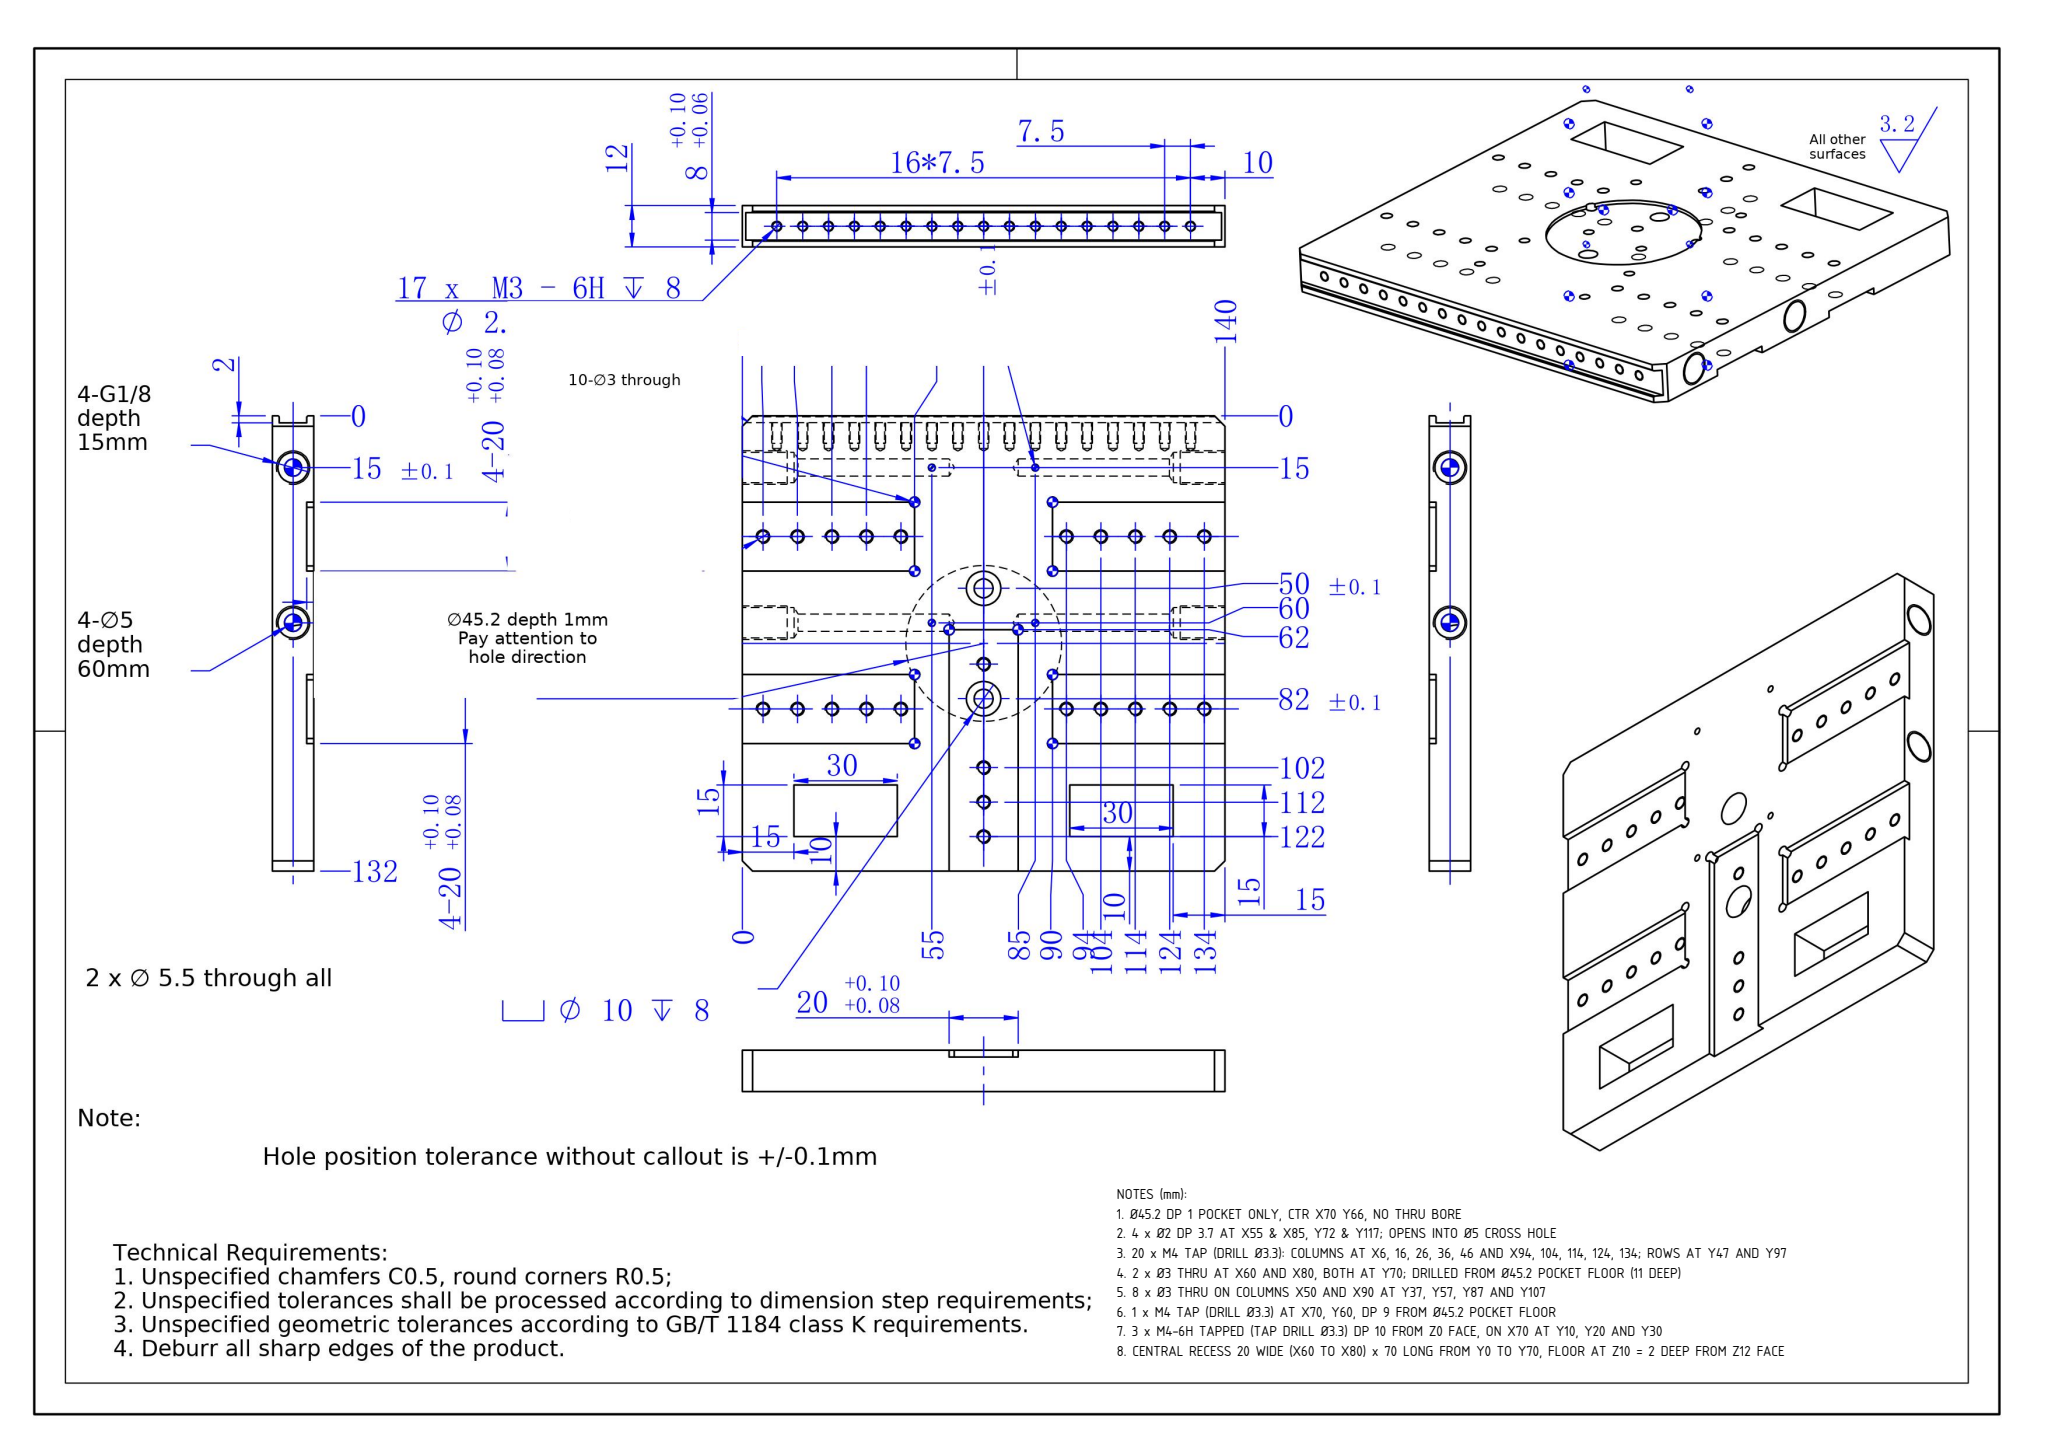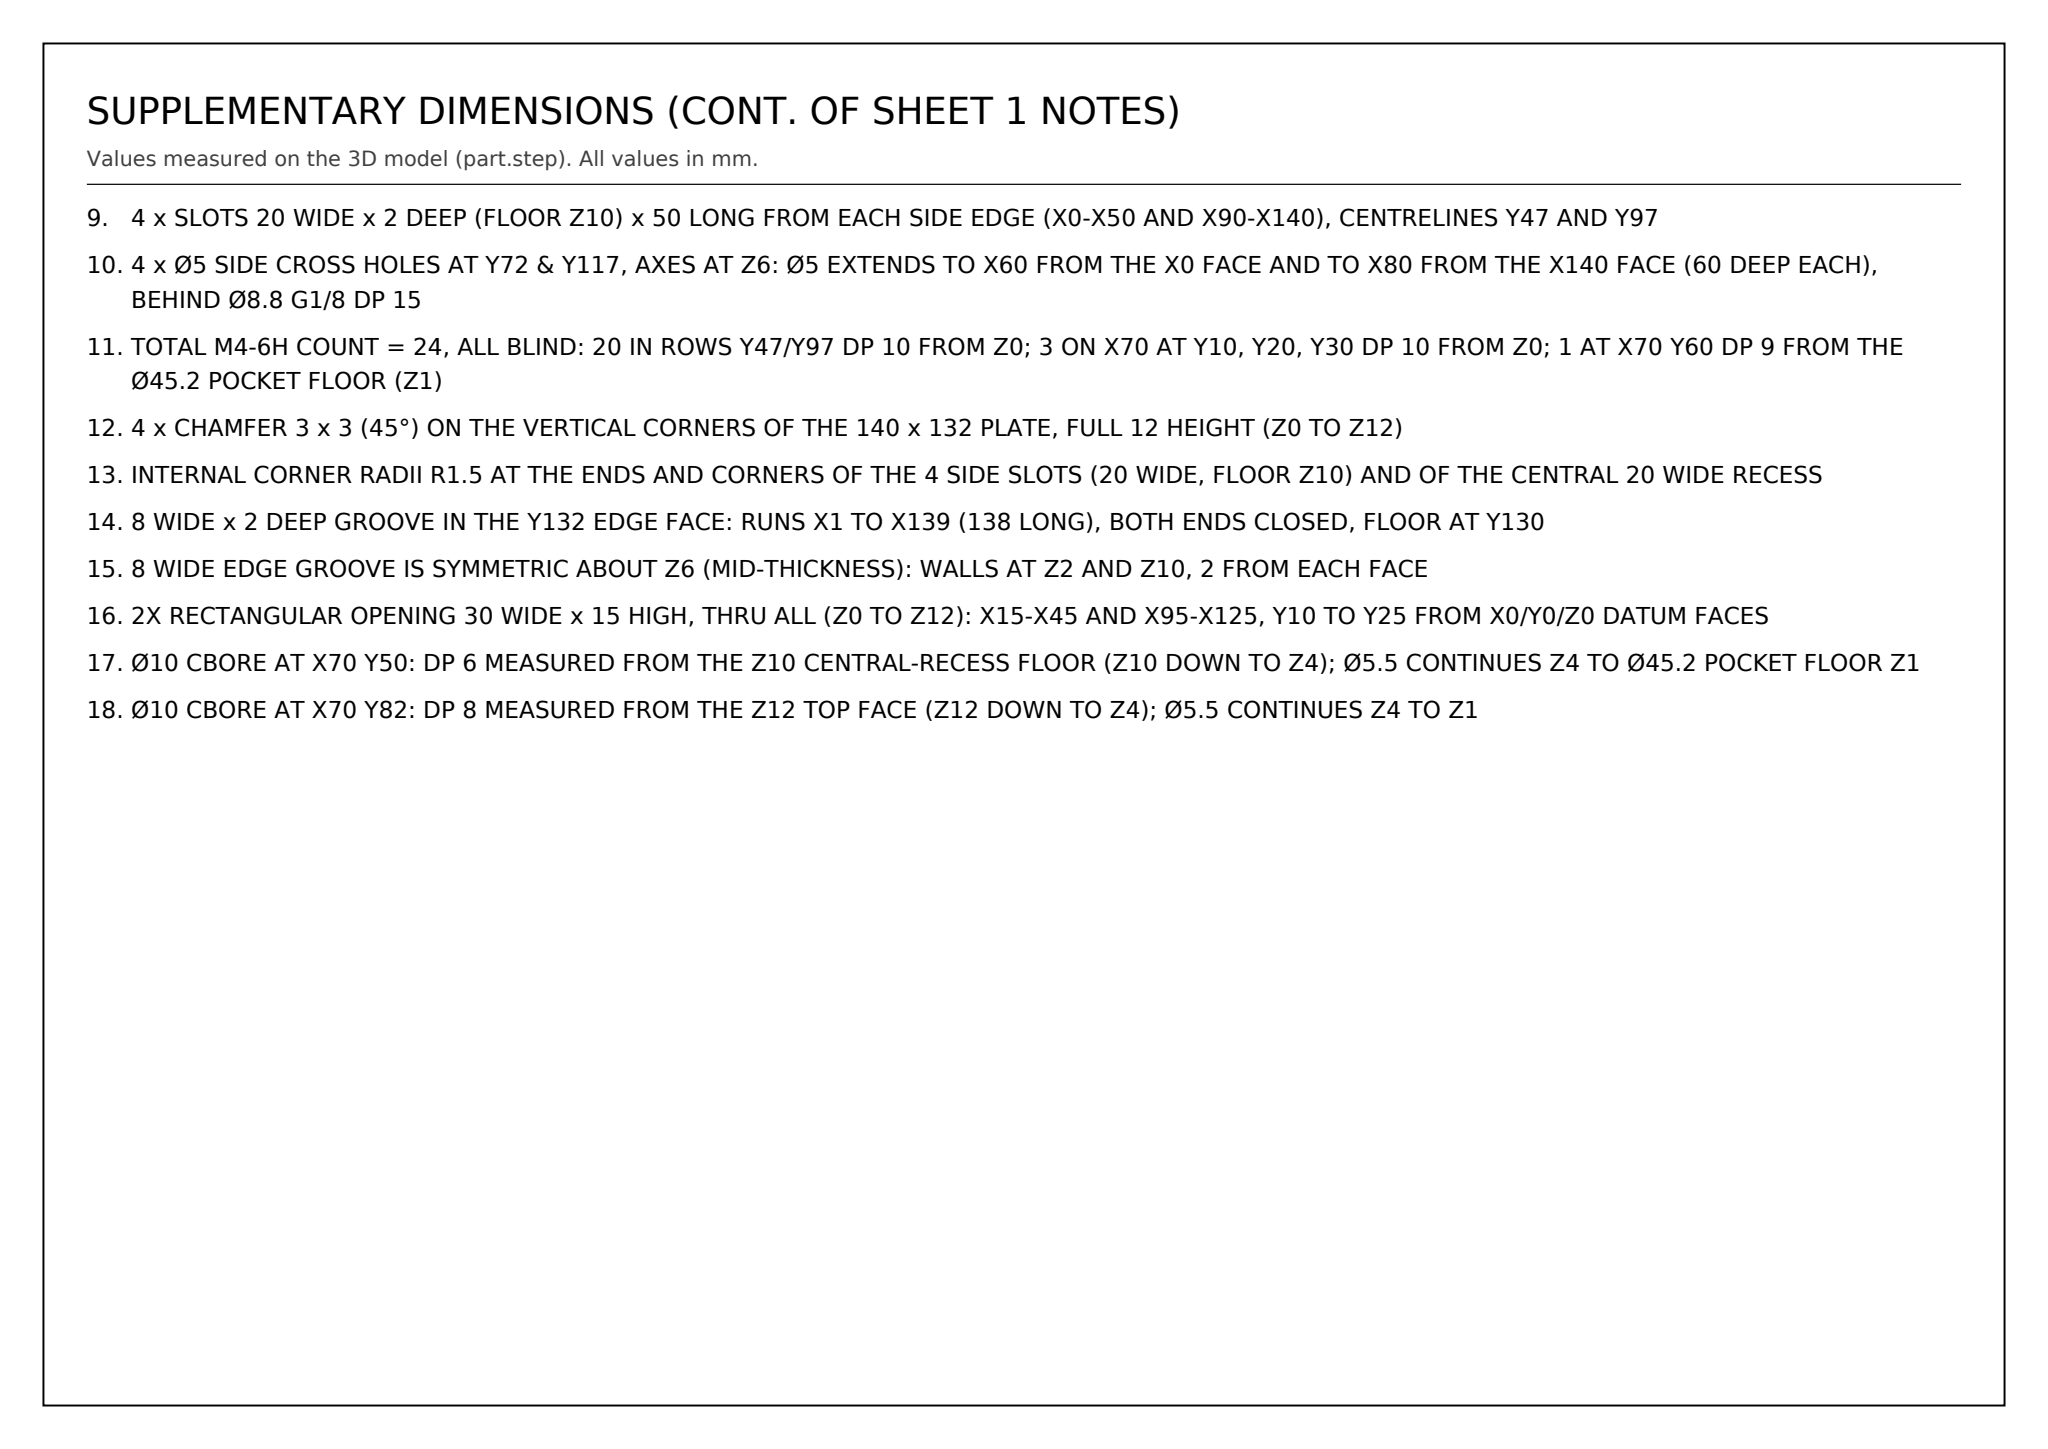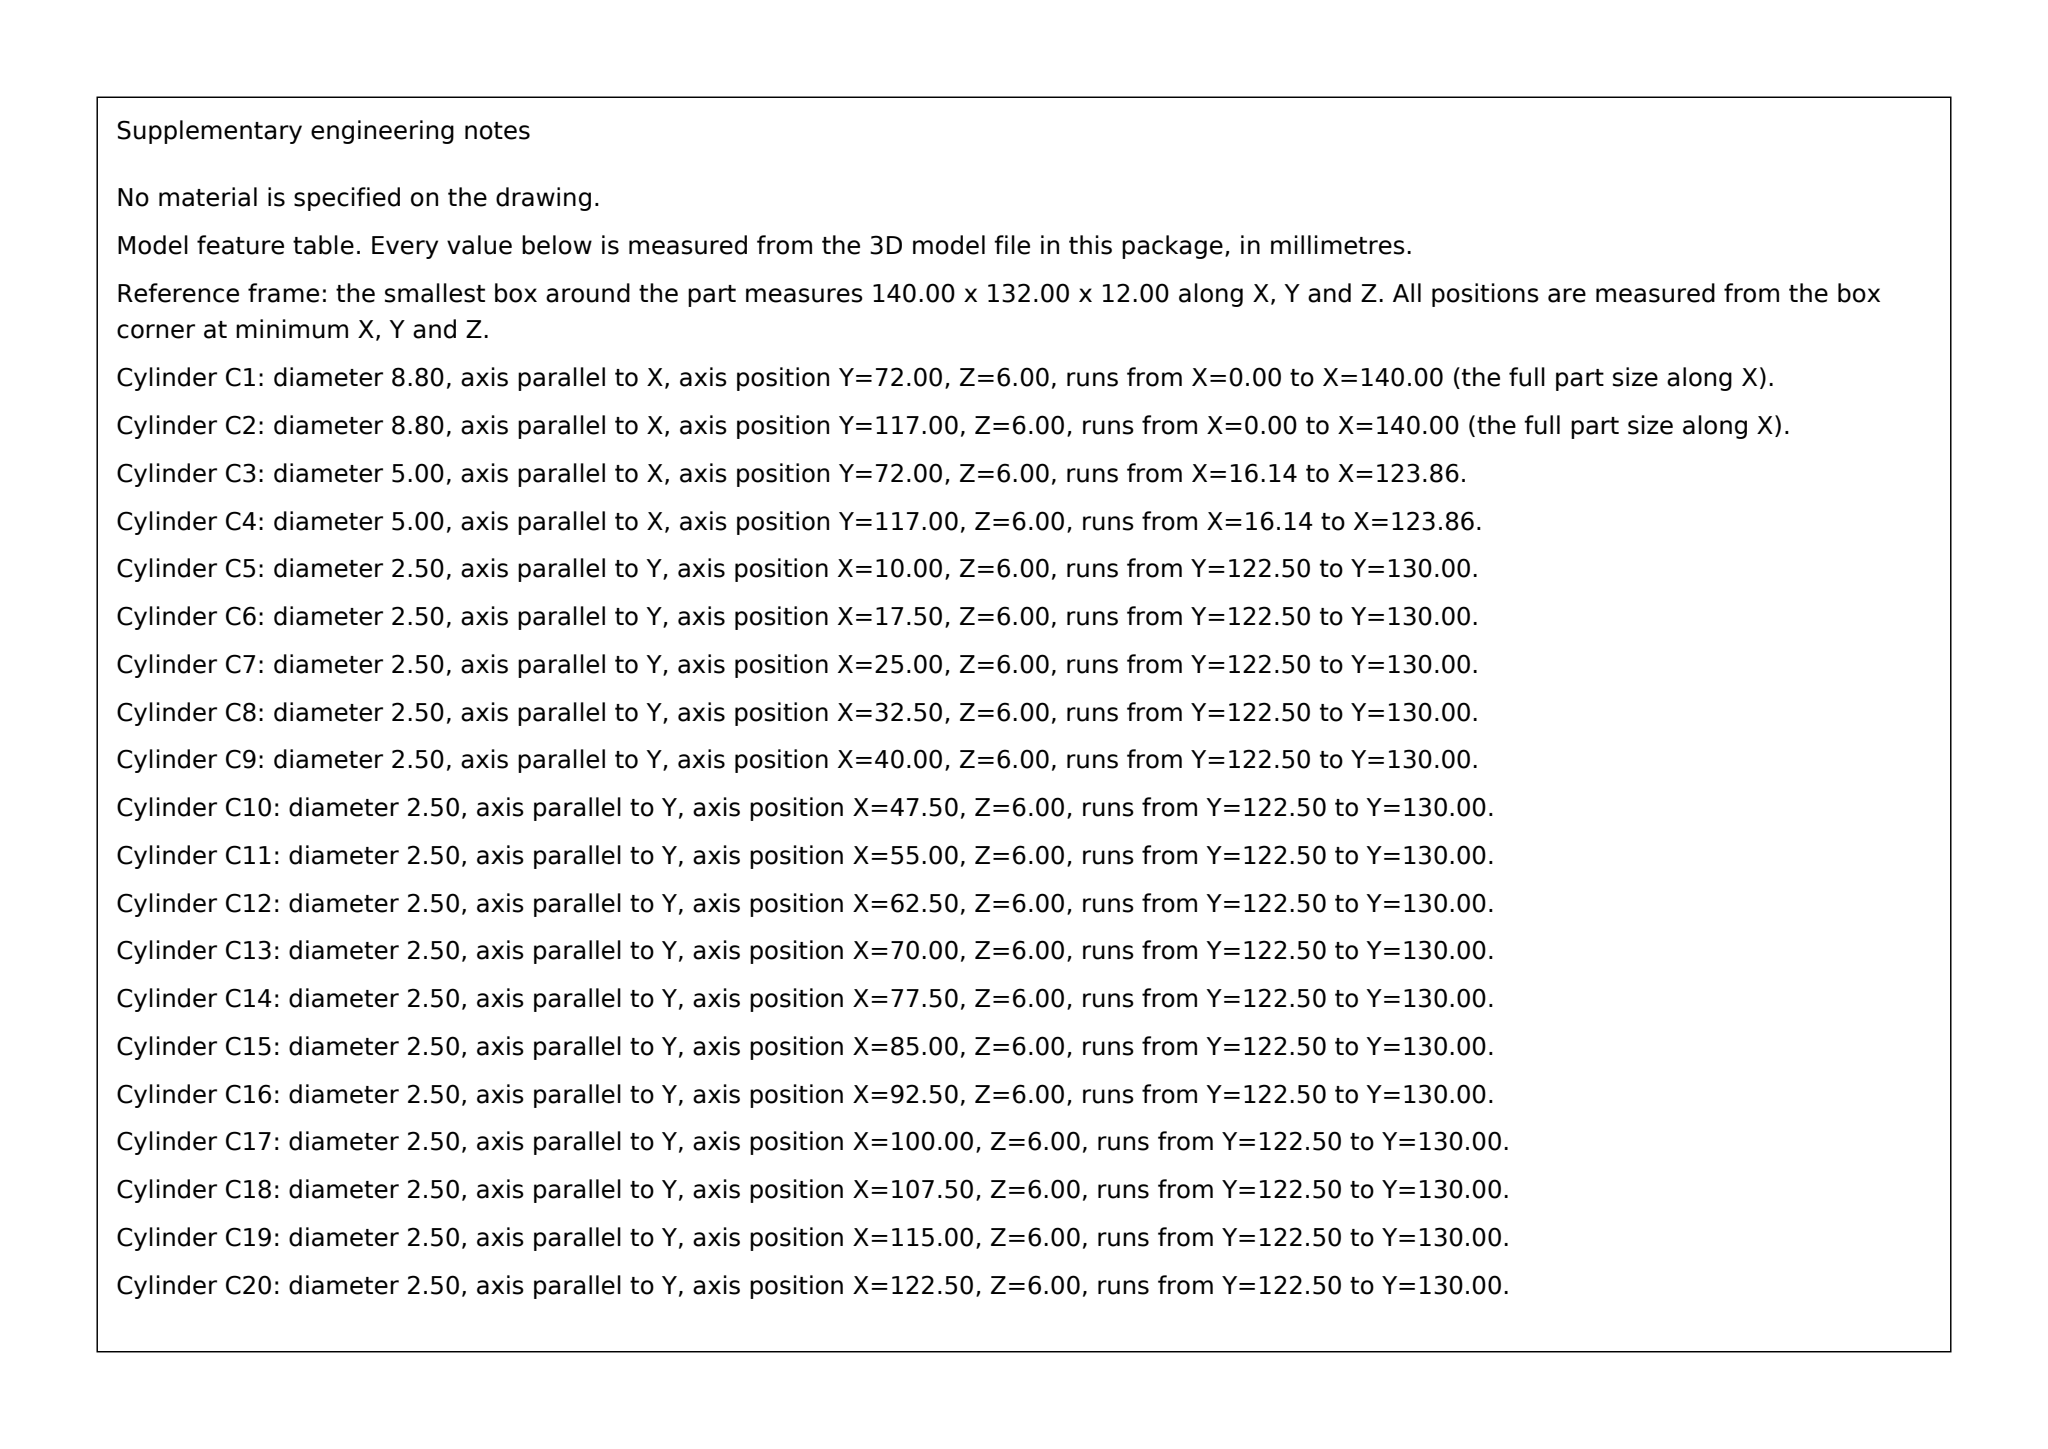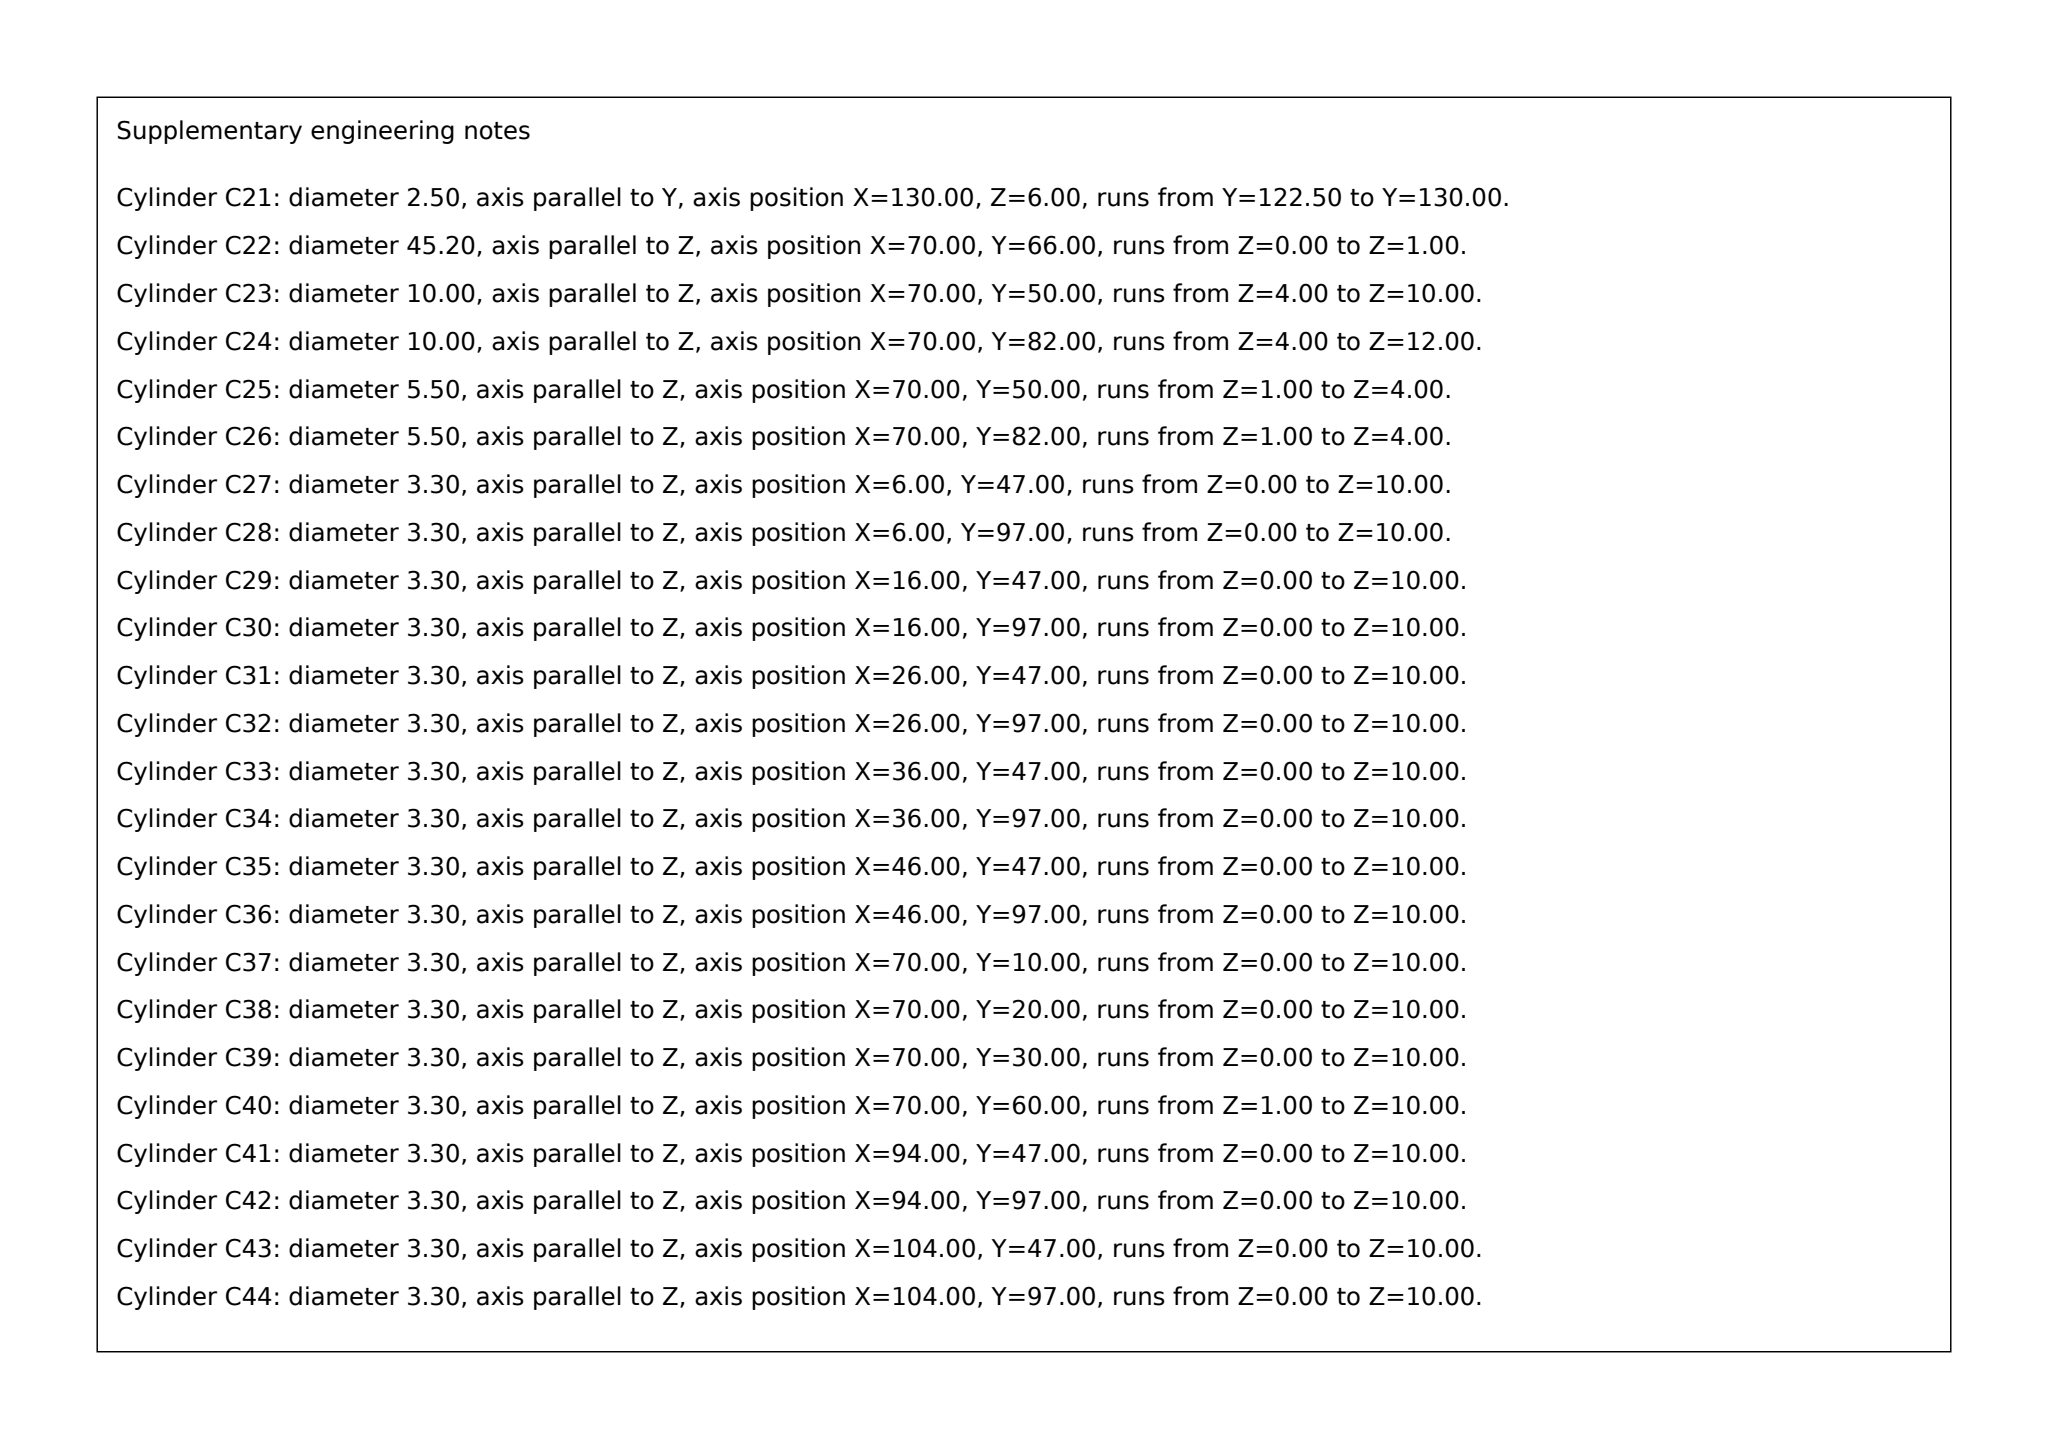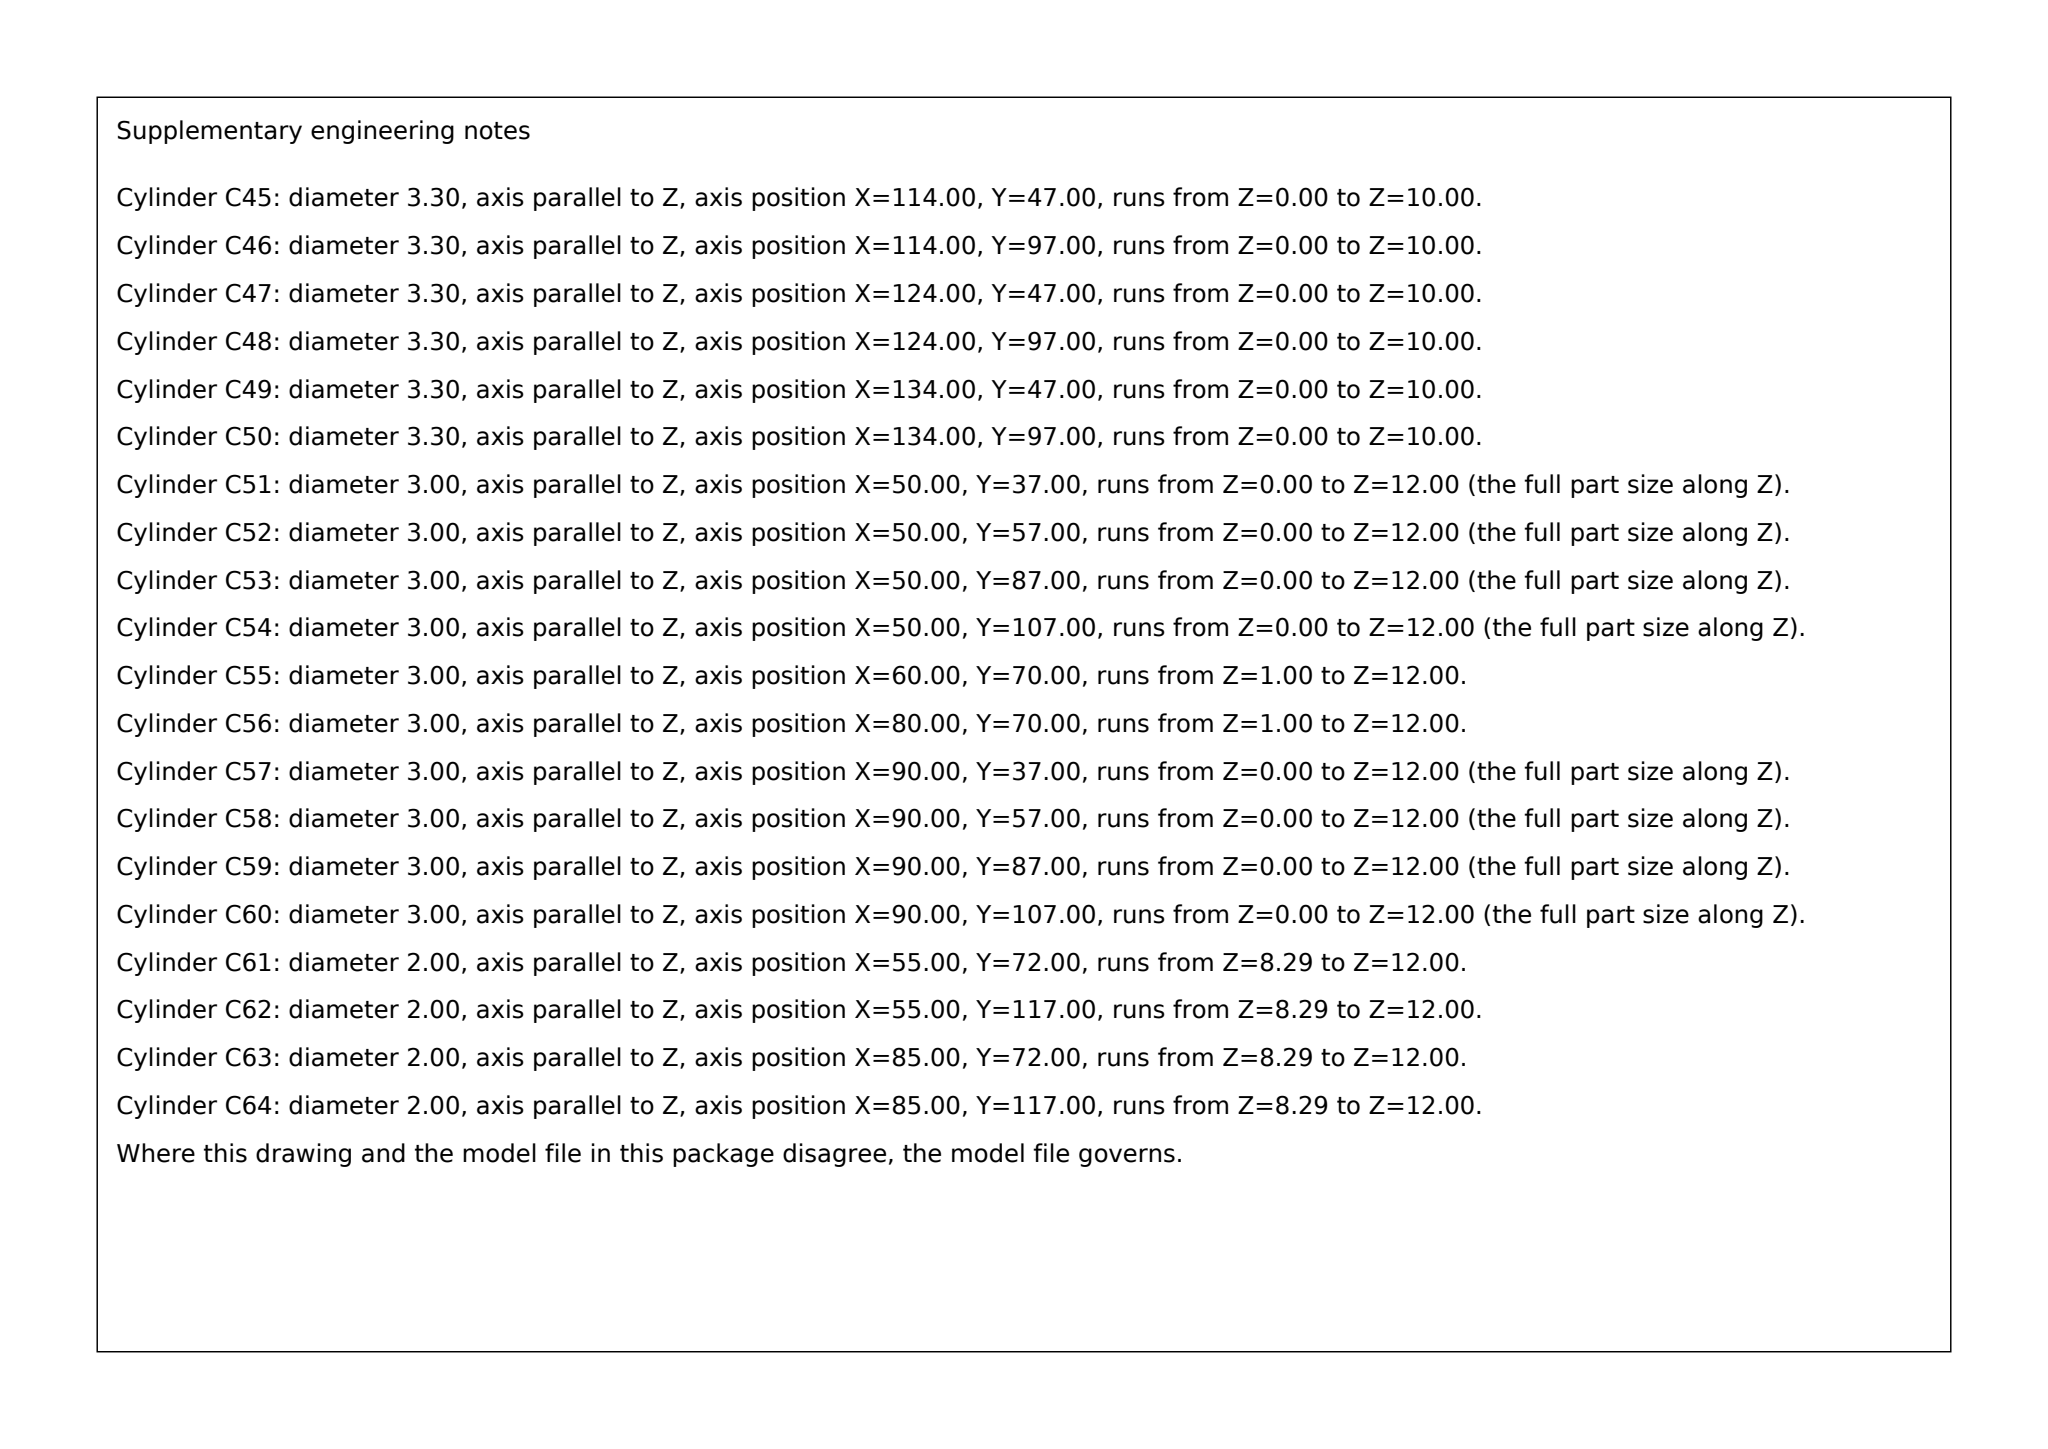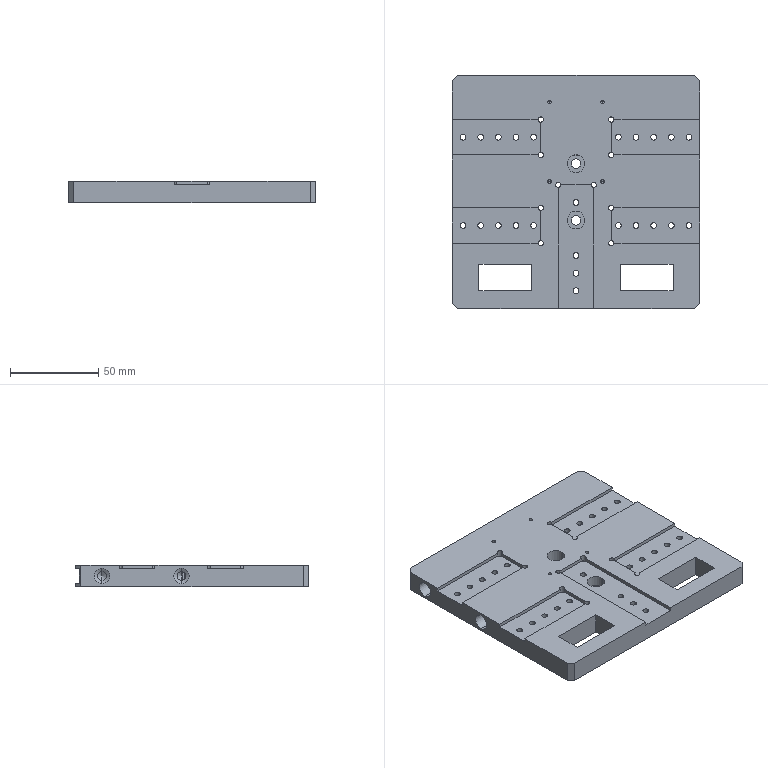Part | SolidWorks | mm | 1 solid | 243 faces | box 140 x 132 x 12 mm | volume 184101 mm3 | cylinder 138 | cone 58 | plane 47 | commonest cylinder face diameters 3.3 x48 2.5 x34 3 x20 8.8 x8 5 x8 2 x8 10 x4 5.5 x4
Drawing notes:
Ø45.2 DP 1 POCKET ONLY, CTR X70 Y66, NO THRU BORE | from the solid: single Ø45.2 z-cyl at (70,66), length 1.0; no larger cylinder in model
4 x Ø2 DP 3.7 AT X55 & X85, Y72 & Y117; OPENS INTO Ø5 CROSS HOLE | from the solid: cylinders Ø2.0 axis z at [55,72],[55,117],[85,72],[85,117], from z8.3 to z12 (3.7 deep from Z12 face); Ø5 cross holes at Y72 & Y117, axis Z6
20 x M4 TAP (DRILL Ø3.3): COLUMNS AT X6, 16, 26, 36, 46 AND X94, 104, 114, 124, 134; ROWS AT Y47 AND Y97 | from the solid: cylinders dia 3.3 axis z at x=6/16/26/36/46 and 94/104/114/124/134, y=47 and 97
2 x Ø3 THRU AT X60 AND X80, BOTH AT Y70; DRILLED FROM Ø45.2 POCKET FLOOR (11 DEEP) | from the solid: cylinders dia 3.0 axis z at (60,70) and (80,70), length 11.0
8 x Ø3 THRU ON COLUMNS X50 AND X90 AT Y37, Y57, Y87 AND Y107 | from the solid: cylinders dia 3.0 axis z at (50,37),(50,57),(50,87),(50,107),(90,37),(90,57),(90,87),(90,107), length 12.0
1 x M4 TAP (DRILL Ø3.3) AT X70, Y60, DP 9 FROM Ø45.2 POCKET FLOOR | from the solid: cylinder dia 3.3 axis z at (70,60), length 9.0
3 x M4-6H TAPPED (TAP DRILL Ø3.3) DP 10 FROM Z0 FACE, ON X70 AT Y10, Y20 AND Y30 | from the solid: cylinders Ø3.3 axis z at (70,10), (70,20), (70,30), from z 0.0 to 10.0
CENTRAL RECESS 20 WIDE (X60 TO X80) x 70 LONG FROM Y0 TO Y70, FLOOR AT Z10 = 2 DEEP FROM Z12 FACE | from the solid: plane normal z at z=10 extent x[60,80] y[0,70]; planes x=60 and x=80 extent y[0,68.5] z[10,12]
4 x SLOTS 20 WIDE x 2 DEEP (FLOOR Z10) x 50 LONG FROM EACH SIDE EDGE (X0-X50 AND X90-X140), CENTRELINES Y47 AND Y97 | from the solid: planes normal z at z=10 extents x[0,50] y[37,57], x[0,50] y[87,107], x[90,140] y[37,57], x[90,140] y[87,107]
4 x Ø5 SIDE CROSS HOLES AT Y72 & Y117, AXES AT Z6: Ø5 EXTENDS TO X60 FROM THE X0 FACE AND TO X80 FROM THE X140 FACE (60 DEEP EACH), BEHIND Ø8.8 G1/8 DP 15 | from the solid: cylinders Ø5.0 axis x at y72/y117, z6, from 16.1 to 60.0 and from 80.0 to 123.9; cylinders Ø8.8 axis x from 0.0 to 15.0 and 125.0 to 140.0
TOTAL M4-6H COUNT = 24, ALL BLIND: 20 IN ROWS Y47/Y97 DP 10 FROM Z0; 3 ON X70 AT Y10, Y20, Y30 DP 10 FROM Z0; 1 AT X70 Y60 DP 9 FROM THE Ø45.2 POCKET FLOOR (Z1) | from the solid: cylinders dia 3.3 axis z: 20 at rows y47/y97 z0-10, 3 at x70 y10/y20/y30 z0-10, 1 at x70 y60 z1-10
4 x CHAMFER 3 x 3 (45°) ON THE VERTICAL CORNERS OF THE 140 x 132 PLATE, FULL 12 HEIGHT (Z0 TO Z12) | from the solid: inclined_planes angle_to_xyz [45,45,90] bbox_from [0,0,0] and [0,129,0] size [3,3,12]; X0/X140 faces extend y3.0-129.0
INTERNAL CORNER RADII R1.5 AT THE ENDS AND CORNERS OF THE 4 SIDE SLOTS (20 WIDE, FLOOR Z10) AND OF THE CENTRAL 20 WIDE RECESS | from the solid: slot end plane x=50 extent y38.5-55.5 inside slot y37-57 (20 wide) and recess end plane x=60 extent y0-68.5 vs floor y0-70, i.e. 1.5 corner relief
8 WIDE x 2 DEEP GROOVE IN THE Y132 EDGE FACE: RUNS X1 TO X139 (138 LONG), BOTH ENDS CLOSED, FLOOR AT Y130 | from the solid: axis_plane y=130 extent x[1.0,139.0] z[2.0,10.0]; z-planes at z2 and z10 extent x[1.0,139.0] y[130,131.7]
8 WIDE EDGE GROOVE IS SYMMETRIC ABOUT Z6 (MID-THICKNESS): WALLS AT Z2 AND Z10, 2 FROM EACH FACE | from the solid: z-planes at z=2.0 and z=10.0, extent x[1,139] y[130,131.7]; bbox thickness z 12
2X RECTANGULAR OPENING 30 WIDE x 15 HIGH, THRU ALL (Z0 TO Z12): X15-X45 AND X95-X125, Y10 TO Y25 FROM X0/Y0/Z0 DATUM FACES | from the solid: axis_planes x=15,45,95,125 each extent y[10,25] z[0,12]; planes y=10 and y=25 extent x[15,45] and x[95,125], z[0,12]
Ø10 CBORE AT X70 Y50: DP 6 MEASURED FROM THE Z10 CENTRAL-RECESS FLOOR (Z10 DOWN TO Z4); Ø5.5 CONTINUES Z4 TO Ø45.2 POCKET FLOOR Z1 | from the solid: cylinder dia 10 axis z at (70,50) from z=4.0 to z=10.0; cylinder dia 5.5 at (70,50) from z=1.0 to z=4.0; plane z=10 extent x[60,80] y[0,70]
Ø10 CBORE AT X70 Y82: DP 8 MEASURED FROM THE Z12 TOP FACE (Z12 DOWN TO Z4); Ø5.5 CONTINUES Z4 TO Z1 | from the solid: cylinder dia 10 axis z at (70,82) from z=4.0 to z=12.0; cylinder dia 5.5 at (70,82) from z=1.0 to z=4.0
build123d program:
from build123d import *

# Parameters (mm, degrees)
SKETCH1_W                                          = 140
SKETCH1_H                                          = 132
BOSS_EXTRUDE1_DEPTH                                = 12
CHAMFER1_SIZE                                      = 3
HOLE_SIZE_ACCORDING_TO_TYPE_OF_HEXAGON_D           = 5.5
HOLE_SIZE_ACCORDING_TO_TYPE_OF_HEXAGON_CBORE_D     = 10
HOLE_SIZE_ACCORDING_TO_TYPE_OF_HEXAGON_CBORE_DEPTH = 8
SKETCH13_R                                         = 22.6
CUT_EXTRUDE3_DEPTH                                 = 1
LPATTERN3_COUNT                                    = 9
LPATTERN3_PITCH                                    = 7.5
LPATTERN3_COL_COUNT                                = 9
LPATTERN3_COL_PITCH                                = 7.5
SKETCH16_W                                         = 140
SKETCH16_H                                         = 8
CUT_EXTRUDE4_DEPTH                                 = 2
CHAMFER2_SIZE                                      = 0.3
SIZE_MM_CLEARANCE_DOWEL_PIN_HOLE_1_D               = 2
SIZE_MM_CLEARANCE_DOWEL_PIN_HOLE_1_DEPTH           = 8
SIZE_MM_CLEARANCE_DOWEL_PIN_HOLE_1_TIP             = 0.6009
SKETCH19_W                                         = 50
SKETCH19_H                                         = 20
CUT_EXTRUDE5_DEPTH                                 = 2
LPATTERN4_COUNT                                    = 2
LPATTERN4_PITCH                                    = 50
MIRROR2_COPY_1_SKETCH_W                            = 50
MIRROR2_COPY_1_SKETCH_H                            = 20
MIRROR2_COPY_1_DEPTH                               = 2
MIRROR2_COPY_2_SKETCH_W                            = 50
MIRROR2_COPY_2_SKETCH_H                            = 20
MIRROR2_COPY_2_DEPTH                               = 2
SKETCH20_W                                         = 20
SKETCH20_H                                         = 70
CUT_EXTRUDE6_DEPTH                                 = 2
SIZE_MM_DOWEL_PIN_HOLE_1_D                         = 3
M4_TAPPED_HOLE1_D                                  = 3.3
M4_TAPPED_HOLE2_D                                  = 3.3
LPATTERN5_COUNT                                    = 5
LPATTERN5_PITCH                                    = 10
LPATTERN6_COUNT                                    = 5
LPATTERN6_PITCH                                    = 10
M4_TAPPED_HOLE3_D                                  = 3.3
LPATTERN7_COUNT                                    = 6
LPATTERN7_PITCH                                    = 10
SIZE_MM_DOWEL_PIN_HOLE_3_D                         = 5
SIZE_MM_DOWEL_PIN_HOLE_3_DEPTH                     = 60
SIZE_MM_DOWEL_PIN_HOLE_3_TIP                       = 1.502
G1_8_TAPPED_HOLE1_D                                = 8.8
G1_8_TAPPED_HOLE1_DEPTH                            = 15
G1_8_TAPPED_HOLE1_TIP                              = 2.644
SIZE_MM_DOWEL_PIN_HOLE_3_2_D                       = 5
SIZE_MM_DOWEL_PIN_HOLE_3_2_DEPTH                   = 60
SIZE_MM_DOWEL_PIN_HOLE_3_2_TIP                     = 1.502
G1_8_TAPPED_HOLE2_D                                = 8.8
G1_8_TAPPED_HOLE2_DEPTH                            = 15
G1_8_TAPPED_HOLE2_TIP                              = 2.644
SKETCH38_W                                         = 30
SKETCH38_H                                         = 15
CUT_EXTRUDE7_DEPTH                                 = 40


with BuildPart() as part:
    # Sketch1 → Boss-Extrude1 (new body)
    with BuildSketch(Plane.XY):
        with Locations((70, 66)):
            Rectangle(SKETCH1_W, SKETCH1_H)
    extrude(amount=BOSS_EXTRUDE1_DEPTH)

    # Chamfer1
    chamfer1_edges = [part.edges().sort_by_distance(p)[0] for p in [
        (0, 132, 6),
        (140, 132, 6),
        (140, 0, 6),
        (0, 0, 6),
    ]]
    chamfer(chamfer1_edges, length=CHAMFER1_SIZE)

    # Hole Size _According to_ Type of Hexagon (through all)
    with Locations(Plane.XY.offset(12)):
        with Locations((70, 82), (70, 50)):
            CounterBoreHole(HOLE_SIZE_ACCORDING_TO_TYPE_OF_HEXAGON_D / 2, HOLE_SIZE_ACCORDING_TO_TYPE_OF_HEXAGON_CBORE_D / 2, HOLE_SIZE_ACCORDING_TO_TYPE_OF_HEXAGON_CBORE_DEPTH)

    # Sketch13 → Cut-Extrude3 (cut)
    with BuildSketch(Plane(origin=(0, 0, 0), x_dir=(-1, 0, 0), z_dir=(0, 0, -1))):
        with Locations((-70, 66)):
            Circle(SKETCH13_R)
    extrude(amount=-CUT_EXTRUDE3_DEPTH, mode=Mode.SUBTRACT)

    # Sketch15 → M3 Tapped Hole1 (revolve, cut)
    with BuildSketch(Plane(origin=(70, 132, 6), x_dir=(0, 0, 1), z_dir=(1, 0, 0))):
        Polygon((0, 0), (0, 10.251), (1.25, 9.5), (1.25, 0), align=None)
    m3_tapped_hole1 = revolve(axis=Axis((70, 138.35, 6), (0, -1, 0)), mode=Mode.SUBTRACT)

    # LPattern3: M3 Tapped Hole1 ×9
    with Locations(*[(-i * LPATTERN3_PITCH, 0, 0) for i in range(1, LPATTERN3_COUNT)]):
        add(m3_tapped_hole1, mode=Mode.SUBTRACT)

    # LPattern3 col: M3 Tapped Hole1 ×9
    with Locations(*[(i * LPATTERN3_COL_PITCH, 0, 0) for i in range(1, LPATTERN3_COL_COUNT)]):
        add(m3_tapped_hole1, mode=Mode.SUBTRACT)

    # Sketch16 → Cut-Extrude4 (cut)
    with BuildSketch(Plane(origin=(0, 132, 0), x_dir=(1, 0, 0), z_dir=(0, 1, 0))):
        with Locations((70, -6)):
            Rectangle(SKETCH16_W, SKETCH16_H)
    extrude(amount=-CUT_EXTRUDE4_DEPTH, mode=Mode.SUBTRACT)

    # Chamfer2
    chamfer2_edges = [part.edges().sort_by_distance(p)[0] for p in [
        (70, 132, 10),
        (70, 132, 2),
    ]]
    chamfer(chamfer2_edges, length=CHAMFER2_SIZE)

    # Size mm Clearance Dowel Pin Hole 1
    with Locations(Plane.XY.offset(12)):
        with Locations((85, 117), (55, 117), (85, 72), (55, 72)):
            Hole(SIZE_MM_CLEARANCE_DOWEL_PIN_HOLE_1_D / 2, depth=SIZE_MM_CLEARANCE_DOWEL_PIN_HOLE_1_DEPTH)
            with Locations((0, 0, -(SIZE_MM_CLEARANCE_DOWEL_PIN_HOLE_1_DEPTH + SIZE_MM_CLEARANCE_DOWEL_PIN_HOLE_1_TIP / 2))):  # 118° drill point
                Cone(0, SIZE_MM_CLEARANCE_DOWEL_PIN_HOLE_1_D / 2, SIZE_MM_CLEARANCE_DOWEL_PIN_HOLE_1_TIP, mode=Mode.SUBTRACT)

    # Sketch19 → Cut-Extrude5 (cut)
    with BuildSketch(Plane.XY.offset(12)):
        with Locations((25, 97)):
            Rectangle(SKETCH19_W, SKETCH19_H)
    cut_extrude5 = extrude(amount=-CUT_EXTRUDE5_DEPTH, mode=Mode.SUBTRACT)

    # Mirror1: Cut-Extrude5 across plane
    add(cut_extrude5.mirror(Plane.ZY.offset(-70)), mode=Mode.SUBTRACT)

    # LPattern4: Cut-Extrude5 ×2
    with Locations(*[(0, -i * LPATTERN4_PITCH, 0) for i in range(1, LPATTERN4_COUNT)]):
        add(cut_extrude5, mode=Mode.SUBTRACT)

    # Mirror2 copy 1 sketch → Mirror2 copy 1 (cut)
    with BuildSketch(Plane(origin=(140, -50, 12), x_dir=(-1, 0, 0), z_dir=(0, 0, 1))):
        with Locations((25, -97)):
            Rectangle(MIRROR2_COPY_1_SKETCH_W, MIRROR2_COPY_1_SKETCH_H)
    extrude(amount=-MIRROR2_COPY_1_DEPTH, mode=Mode.SUBTRACT)

    # Mirror2 copy 2 sketch → Mirror2 copy 2 (cut)
    with BuildSketch(Plane(origin=(140, 0, 12), x_dir=(-1, 0, 0), z_dir=(0, 0, 1))):
        with Locations((25, -97)):
            Rectangle(MIRROR2_COPY_2_SKETCH_W, MIRROR2_COPY_2_SKETCH_H)
    extrude(amount=-MIRROR2_COPY_2_DEPTH, mode=Mode.SUBTRACT)

    # Sketch20 → Cut-Extrude6 (cut)
    with BuildSketch(Plane.XY.offset(12)):
        with Locations((70, 35)):
            Rectangle(SKETCH20_W, SKETCH20_H)
    extrude(amount=-CUT_EXTRUDE6_DEPTH, mode=Mode.SUBTRACT)

    # Size mm Dowel Pin Hole 1 (through all)
    with Locations(Plane.XY.offset(12)):
        with Locations((50, 87), (50, 107), (50, 37), (50, 57), (90, 87), (90, 107), (90, 37), (90, 57), (60, 70), (80, 70)):
            Hole(SIZE_MM_DOWEL_PIN_HOLE_1_D / 2)

    # M4 Tapped Hole1 (through all)
    with Locations(Plane.XY.offset(10)):
        with Locations((46, 97), (46, 47)):
            m4_tapped_hole1 = Hole(M4_TAPPED_HOLE1_D / 2)

    # M4 Tapped Hole2 (through all)
    with Locations(Plane.XY.offset(10)):
        with Locations((94, 97), (94, 47)):
            m4_tapped_hole2 = Hole(M4_TAPPED_HOLE2_D / 2)

    # LPattern5: M4 Tapped Hole1 ×5
    with Locations(*[(-i * LPATTERN5_PITCH, 0, 0) for i in range(1, LPATTERN5_COUNT)]):
        add(m4_tapped_hole1, mode=Mode.SUBTRACT)

    # LPattern6: M4 Tapped Hole2 ×5
    with Locations(*[(i * LPATTERN6_PITCH, 0, 0) for i in range(1, LPATTERN6_COUNT)]):
        add(m4_tapped_hole2, mode=Mode.SUBTRACT)

    # M4 Tapped Hole3 (through all)
    with Locations(Plane.XY.offset(10)):
        with Locations((70, 10)):
            m4_tapped_hole3 = Hole(M4_TAPPED_HOLE3_D / 2)

    # LPattern7: M4 Tapped Hole3 ×6, 1 skipped
    with Locations(*[(0, i * LPATTERN7_PITCH, 0) for i in range(1, LPATTERN7_COUNT) if i not in (3,)]):
        add(m4_tapped_hole3, mode=Mode.SUBTRACT)

    # Size mm Dowel Pin Hole 3
    with Locations(Plane.ZY):
        with Locations((6, 117), (6, 72)):
            Hole(SIZE_MM_DOWEL_PIN_HOLE_3_D / 2, depth=SIZE_MM_DOWEL_PIN_HOLE_3_DEPTH)
            with Locations((0, 0, -(SIZE_MM_DOWEL_PIN_HOLE_3_DEPTH + SIZE_MM_DOWEL_PIN_HOLE_3_TIP / 2))):  # 118° drill point
                Cone(0, SIZE_MM_DOWEL_PIN_HOLE_3_D / 2, SIZE_MM_DOWEL_PIN_HOLE_3_TIP, mode=Mode.SUBTRACT)

    # G1_8 Tapped Hole1
    with Locations(Plane.ZY):
        with Locations((6, 117), (6, 72)):
            Hole(G1_8_TAPPED_HOLE1_D / 2, depth=G1_8_TAPPED_HOLE1_DEPTH)
            with Locations((0, 0, -(G1_8_TAPPED_HOLE1_DEPTH + G1_8_TAPPED_HOLE1_TIP / 2))):  # 118° drill point
                Cone(0, G1_8_TAPPED_HOLE1_D / 2, G1_8_TAPPED_HOLE1_TIP, mode=Mode.SUBTRACT)

    # Size mm Dowel Pin Hole 3_2
    with Locations(Plane(origin=(140, 0, 0), x_dir=(0, 0, -1), z_dir=(1, 0, 0))):
        with Locations((-6, 117), (-6, 72)):
            Hole(SIZE_MM_DOWEL_PIN_HOLE_3_2_D / 2, depth=SIZE_MM_DOWEL_PIN_HOLE_3_2_DEPTH)
            with Locations((0, 0, -(SIZE_MM_DOWEL_PIN_HOLE_3_2_DEPTH + SIZE_MM_DOWEL_PIN_HOLE_3_2_TIP / 2))):  # 118° drill point
                Cone(0, SIZE_MM_DOWEL_PIN_HOLE_3_2_D / 2, SIZE_MM_DOWEL_PIN_HOLE_3_2_TIP, mode=Mode.SUBTRACT)

    # G1_8 Tapped Hole2
    with Locations(Plane(origin=(140, 0, 0), x_dir=(0, 0, -1), z_dir=(1, 0, 0))):
        with Locations((-6, 117), (-6, 72)):
            Hole(G1_8_TAPPED_HOLE2_D / 2, depth=G1_8_TAPPED_HOLE2_DEPTH)
            with Locations((0, 0, -(G1_8_TAPPED_HOLE2_DEPTH + G1_8_TAPPED_HOLE2_TIP / 2))):  # 118° drill point
                Cone(0, G1_8_TAPPED_HOLE2_D / 2, G1_8_TAPPED_HOLE2_TIP, mode=Mode.SUBTRACT)

    # Sketch38 → Cut-Extrude7 (cut)
    with BuildSketch(Plane.XY.offset(12)):
        with Locations((30, 17.5)):
            Rectangle(SKETCH38_W, SKETCH38_H)
        with Locations((110, 17.5)):
            Rectangle(SKETCH38_W, SKETCH38_H)
    extrude(amount=-CUT_EXTRUDE7_DEPTH, mode=Mode.SUBTRACT)


solid = part.part